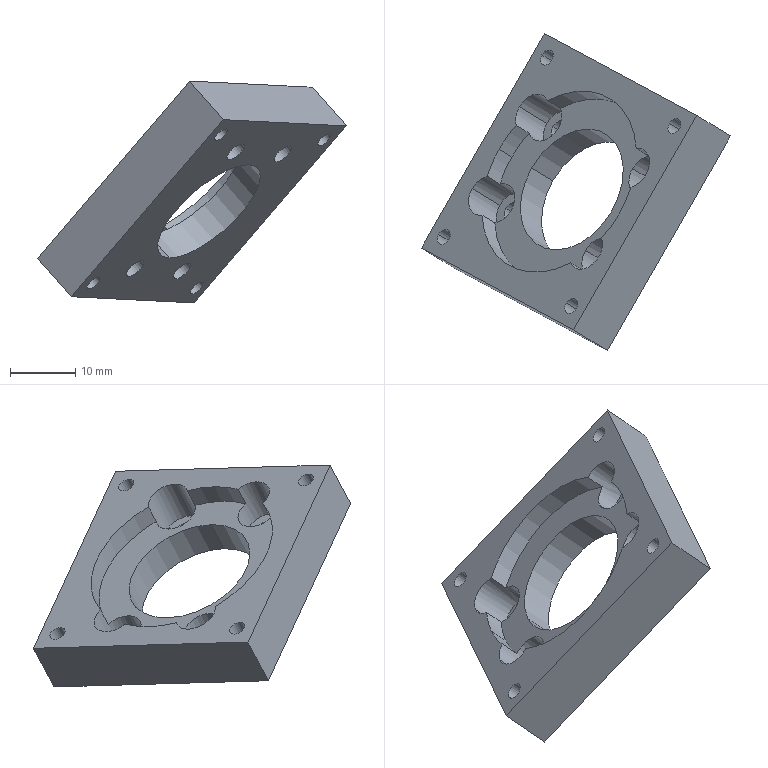Component | SolidWorks | KK40-100A1-F0z0-123-2_f2z0-123-1 | 1 solid | 42 faces | box 47.47 x 48.72 x 34.08 mm | volume 7450 mm3 | cylinder 31 | plane 11 | commonest cylinder face diameters 3.4 x8 6.5 x8 2.5 x8 30 x5 20 x2
build123d program:
from build123d import *

# Parameters (mm, degrees)
SKETCH1_W                                       = 38
SKETCH1_H                                       = 38
BOSS_EXTRUDE1_DEPTH                             = 8.5
SKETCH2_R                                       = 15
CUT_EXTRUDE1_DEPTH                              = 3.2
SKETCH3_R                                       = 10
CUT_EXTRUDE2_DEPTH                              = 28.388
M3_TAPPED_HOLE1_D                               = 2.5
M3_TAPPED_HOLE1_DEPTH                           = 18
M3_TAPPED_HOLE1_TIP                             = 0.7511
M3_HEX_SOCKET_HEAD_CAP_SCREW_CBORE1_D           = 3.4
M3_HEX_SOCKET_HEAD_CAP_SCREW_CBORE1_CBORE_D     = 6.5
M3_HEX_SOCKET_HEAD_CAP_SCREW_CBORE1_CBORE_DEPTH = 6.9


with BuildPart() as part:
    # Sketch1 → Boss-Extrude1 (new body)
    with BuildSketch(Plane.XY):
        Rectangle(SKETCH1_W, SKETCH1_H)
    extrude(amount=BOSS_EXTRUDE1_DEPTH)

    # Sketch2 → Cut-Extrude1 (cut)
    with BuildSketch(Plane.XY.offset(8.5)):
        Circle(SKETCH2_R)
    extrude(amount=-CUT_EXTRUDE1_DEPTH, mode=Mode.SUBTRACT)

    # Sketch3 → Cut-Extrude2 (cut, through all)
    with BuildSketch(Plane.XY.offset(5.3)):
        Circle(SKETCH3_R)
    extrude(amount=-CUT_EXTRUDE2_DEPTH, mode=Mode.SUBTRACT)

    # M3 Tapped Hole1
    with Locations(Plane.XY.offset(8.5)):
        with Locations((-15.91, 15.91), (15.91, 15.91), (15.91, -15.91), (-15.91, -15.91)):
            Hole(M3_TAPPED_HOLE1_D / 2, depth=M3_TAPPED_HOLE1_DEPTH)
            with Locations((0, 0, -(M3_TAPPED_HOLE1_DEPTH + M3_TAPPED_HOLE1_TIP / 2))):  # 118° drill point
                Cone(0, M3_TAPPED_HOLE1_D / 2, M3_TAPPED_HOLE1_TIP, mode=Mode.SUBTRACT)

    # M3 Hex Socket Head Cap Screw CBORE1 (through all)
    with Locations(Plane.XY.offset(8.5)):
        with Locations((-12.557, 7.25), (12.557, 7.25), (12.557, -7.25), (-12.557, -7.25)):
            CounterBoreHole(M3_HEX_SOCKET_HEAD_CAP_SCREW_CBORE1_D / 2, M3_HEX_SOCKET_HEAD_CAP_SCREW_CBORE1_CBORE_D / 2, M3_HEX_SOCKET_HEAD_CAP_SCREW_CBORE1_CBORE_DEPTH)


solid = part.part

# Placed as in the assembly
solid = solid.moved(Location((5.226, 16.243, 239.026), (-28.021, -37.728, -38.997)))